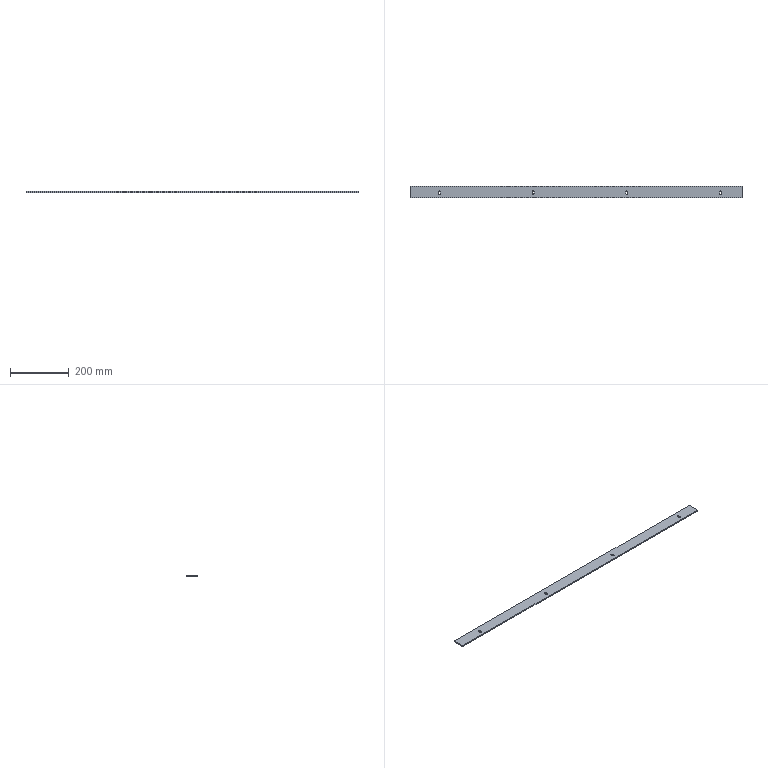Component | SolidWorks | SlideRail-1 | 1 solid | 22 faces | box 1133 x 40 x 4 mm | volume 180104 mm3 | plane 14 | cylinder 8 | commonest cylinder face diameters 7 x8
build123d program:
from build123d import *

# Parameters (mm, degrees)
SKETCH1_W           = 1133
SKETCH1_H           = 40
BOSS_EXTRUDE1_DEPTH = 4
CUT_EXTRUDE1_DEPTH  = 10
LPATTERN1_COUNT     = 4
LPATTERN1_PITCH     = 320


with BuildPart() as part:
    # Sketch1 → Boss-Extrude1 (new body)
    with BuildSketch(Plane.XY):
        with Locations((460.15, 15.317)):
            Rectangle(SKETCH1_W, SKETCH1_H)
    extrude(amount=BOSS_EXTRUDE1_DEPTH)

    # Sketch2 → Cut-Extrude1 (cut)
    with BuildSketch(Plane.XY.offset(4)):
        with BuildLine():
            Line((-2.85, 15.317), (-2.85, 10.317))
            ThreePointArc((-2.85, 10.317), (-6.35, 6.817), (-9.85, 10.317))
            Line((-9.85, 10.317), (-9.85, 15.317))
            ThreePointArc((-9.85, 15.317), (-6.35, 18.817), (-2.85, 15.317))
        make_face()
    cut_extrude1 = extrude(amount=-CUT_EXTRUDE1_DEPTH, mode=Mode.SUBTRACT)

    # LPattern1: Cut-Extrude1 ×4
    with Locations(*[(i * LPATTERN1_PITCH, 0, 0) for i in range(1, LPATTERN1_COUNT)]):
        add(cut_extrude1, mode=Mode.SUBTRACT)


solid = part.part

# Placed as in the assembly
solid = solid.moved(Location((-791.2, -396.75, 487.481), (0, 0, 0)))
STEP:
#1=COLOUR_RGB('',0.7922,0.8196,0.9333);
#2=FILL_AREA_STYLE_COLOUR('',#1);
#3=FILL_AREA_STYLE('',(#2));
#4=SURFACE_STYLE_FILL_AREA(#3);
#5=SURFACE_SIDE_STYLE('',(#4));
#6=SURFACE_STYLE_USAGE(.BOTH.,#5);
#7=PRESENTATION_STYLE_ASSIGNMENT((#6));
#8=CARTESIAN_POINT('',(-35.337,-14.23,19.192));
#9=VERTEX_POINT('',#8);
#10=CARTESIAN_POINT('',(-35.337,-15.804,19.192));
#11=VERTEX_POINT('',#10);
#12=CARTESIAN_POINT('',(-35.337,-14.23,19.192));
#13=DIRECTION('',(0.,-1.,0.));
#14=VECTOR('',#13,39.37);
#15=LINE('',#12,#14);
#16=EDGE_CURVE('',#9,#11,#15,.T.);
#17=ORIENTED_EDGE('',*,*,#16,.T.);
#18=CARTESIAN_POINT('',(-35.337,-15.804,19.35));
#19=VERTEX_POINT('',#18);
#20=CARTESIAN_POINT('',(-35.337,-15.804,19.35));
#21=DIRECTION('',(0.,0.,-1.));
#22=VECTOR('',#21,39.37);
#23=LINE('',#20,#22);
#24=EDGE_CURVE('',#19,#11,#23,.T.);
#25=ORIENTED_EDGE('',*,*,#24,.F.);
#26=CARTESIAN_POINT('',(-35.337,-14.23,19.35));
#27=VERTEX_POINT('',#26);
#28=CARTESIAN_POINT('',(-35.337,-14.23,19.35));
#29=DIRECTION('',(0.,-1.,0.));
#30=VECTOR('',#29,39.37);
#31=LINE('',#28,#30);
#32=EDGE_CURVE('',#27,#19,#31,.T.);
#33=ORIENTED_EDGE('',*,*,#32,.F.);
#34=CARTESIAN_POINT('',(-35.337,-14.23,19.35));
#35=DIRECTION('',(0.,0.,-1.));
#36=VECTOR('',#35,39.37);
#37=LINE('',#34,#36);
#38=EDGE_CURVE('',#27,#9,#37,.T.);
#39=ORIENTED_EDGE('',*,*,#38,.T.);
#40=EDGE_LOOP('',(#17,#25,#33,#39));
#41=FACE_OUTER_BOUND('',#40,.T.);
#42=CARTESIAN_POINT('',(-35.337,-14.23,19.35));
#43=DIRECTION('',(1.,0.,0.));
#44=DIRECTION('',(0.,0.,-1.));
#45=AXIS2_PLACEMENT_3D('',#42,#43,#44);
#46=PLANE('',#45);
#47=ADVANCED_FACE('',(#41),#46,.F.);
#48=CARTESIAN_POINT('',(9.27,-15.804,19.192));
#49=VERTEX_POINT('',#48);
#50=CARTESIAN_POINT('',(-35.337,-15.804,19.192));
#51=DIRECTION('',(1.,-0.,0.));
#52=VECTOR('',#51,39.37);
#53=LINE('',#50,#52);
#54=EDGE_CURVE('',#11,#49,#53,.T.);
#55=ORIENTED_EDGE('',*,*,#54,.T.);
#56=CARTESIAN_POINT('',(9.27,-15.804,19.35));
#57=VERTEX_POINT('',#56);
#58=CARTESIAN_POINT('',(9.27,-15.804,19.35));
#59=DIRECTION('',(0.,0.,-1.));
#60=VECTOR('',#59,39.37);
#61=LINE('',#58,#60);
#62=EDGE_CURVE('',#57,#49,#61,.T.);
#63=ORIENTED_EDGE('',*,*,#62,.F.);
#64=CARTESIAN_POINT('',(-35.337,-15.804,19.35));
#65=DIRECTION('',(1.,-0.,0.));
#66=VECTOR('',#65,39.37);
#67=LINE('',#64,#66);
#68=EDGE_CURVE('',#19,#57,#67,.T.);
#69=ORIENTED_EDGE('',*,*,#68,.F.);
#70=ORIENTED_EDGE('',*,*,#24,.T.);
#71=EDGE_LOOP('',(#55,#63,#69,#70));
#72=FACE_OUTER_BOUND('',#71,.T.);
#73=CARTESIAN_POINT('',(-35.337,-15.804,19.35));
#74=DIRECTION('',(0.,1.,0.));
#75=DIRECTION('',(-1.,0.,0.));
#76=AXIS2_PLACEMENT_3D('',#73,#74,#75);
#77=PLANE('',#76);
#78=ADVANCED_FACE('',(#72),#77,.F.);
#79=CARTESIAN_POINT('',(9.27,-14.23,19.192));
#80=VERTEX_POINT('',#79);
#81=CARTESIAN_POINT('',(9.27,-14.23,19.192));
#82=DIRECTION('',(0.,1.,0.));
#83=VECTOR('',#82,39.37);
#84=LINE('',#81,#83);
#85=EDGE_CURVE('',#49,#80,#84,.T.);
#86=ORIENTED_EDGE('',*,*,#85,.T.);
#87=CARTESIAN_POINT('',(9.27,-14.23,19.35));
#88=VERTEX_POINT('',#87);
#89=CARTESIAN_POINT('',(9.27,-14.23,19.35));
#90=DIRECTION('',(0.,0.,-1.));
#91=VECTOR('',#90,39.37);
#92=LINE('',#89,#91);
#93=EDGE_CURVE('',#88,#80,#92,.T.);
#94=ORIENTED_EDGE('',*,*,#93,.F.);
#95=CARTESIAN_POINT('',(9.27,-14.23,19.35));
#96=DIRECTION('',(0.,1.,0.));
#97=VECTOR('',#96,39.37);
#98=LINE('',#95,#97);
#99=EDGE_CURVE('',#57,#88,#98,.T.);
#100=ORIENTED_EDGE('',*,*,#99,.F.);
#101=ORIENTED_EDGE('',*,*,#62,.T.);
#102=EDGE_LOOP('',(#86,#94,#100,#101));
#103=FACE_OUTER_BOUND('',#102,.T.);
#104=CARTESIAN_POINT('',(9.27,-14.23,19.35));
#105=DIRECTION('',(-1.,0.,0.));
#106=DIRECTION('',(0.,0.,1.));
#107=AXIS2_PLACEMENT_3D('',#104,#105,#106);
#108=PLANE('',#107);
#109=ADVANCED_FACE('',(#103),#108,.F.);
#110=CARTESIAN_POINT('',(-35.337,-14.23,19.192));
#111=DIRECTION('',(-1.,0.,0.));
#112=VECTOR('',#111,39.37);
#113=LINE('',#110,#112);
#114=EDGE_CURVE('',#80,#9,#113,.T.);
#115=ORIENTED_EDGE('',*,*,#114,.T.);
#116=ORIENTED_EDGE('',*,*,#38,.F.);
#117=CARTESIAN_POINT('',(-35.337,-14.23,19.35));
#118=DIRECTION('',(-1.,0.,0.));
#119=VECTOR('',#118,39.37);
#120=LINE('',#117,#119);
#121=EDGE_CURVE('',#88,#27,#120,.T.);
#122=ORIENTED_EDGE('',*,*,#121,.F.);
#123=ORIENTED_EDGE('',*,*,#93,.T.);
#124=EDGE_LOOP('',(#115,#116,#122,#123));
#125=FACE_OUTER_BOUND('',#124,.T.);
#126=CARTESIAN_POINT('',(-35.337,-14.23,19.35));
#127=DIRECTION('',(0.,-1.,0.));
#128=DIRECTION('',(0.,0.,-1.));
#129=AXIS2_PLACEMENT_3D('',#126,#127,#128);
#130=PLANE('',#129);
#131=ADVANCED_FACE('',(#125),#130,.F.);
#132=CARTESIAN_POINT('',(-18.663,-15.017,19.35));
#133=VERTEX_POINT('',#132);
#134=CARTESIAN_POINT('',(-18.939,-15.017,19.35));
#135=VERTEX_POINT('',#134);
#136=CARTESIAN_POINT('',(-18.801,-15.017,19.35));
#137=DIRECTION('',(0.,0.,1.));
#138=DIRECTION('',(1.,0.,0.));
#139=AXIS2_PLACEMENT_3D('',#136,#137,#138);
#140=CIRCLE('',#139,0.1378);
#141=EDGE_CURVE('',#133,#135,#140,.T.);
#142=ORIENTED_EDGE('',*,*,#141,.F.);
#143=CARTESIAN_POINT('',(-18.663,-15.214,19.35));
#144=VERTEX_POINT('',#143);
#145=CARTESIAN_POINT('',(-18.663,-15.017,19.35));
#146=DIRECTION('',(0.,1.,0.));
#147=VECTOR('',#146,39.37);
#148=LINE('',#145,#147);
#149=EDGE_CURVE('',#144,#133,#148,.T.);
#150=ORIENTED_EDGE('',*,*,#149,.F.);
#151=CARTESIAN_POINT('',(-18.939,-15.214,19.35));
#152=VERTEX_POINT('',#151);
#153=CARTESIAN_POINT('',(-18.801,-15.214,19.35));
#154=DIRECTION('',(0.,0.,1.));
#155=DIRECTION('',(1.,0.,0.));
#156=AXIS2_PLACEMENT_3D('',#153,#154,#155);
#157=CIRCLE('',#156,0.1378);
#158=EDGE_CURVE('',#152,#144,#157,.T.);
#159=ORIENTED_EDGE('',*,*,#158,.F.);
#160=CARTESIAN_POINT('',(-18.939,-15.017,19.35));
#161=DIRECTION('',(0.,-1.,0.));
#162=VECTOR('',#161,39.37);
#163=LINE('',#160,#162);
#164=EDGE_CURVE('',#135,#152,#163,.T.);
#165=ORIENTED_EDGE('',*,*,#164,.F.);
#166=EDGE_LOOP('',(#142,#150,#159,#165));
#167=FACE_BOUND('',#166,.T.);
#168=CARTESIAN_POINT('',(-31.262,-15.017,19.35));
#169=VERTEX_POINT('',#168);
#170=CARTESIAN_POINT('',(-31.537,-15.017,19.35));
#171=VERTEX_POINT('',#170);
#172=CARTESIAN_POINT('',(-31.4,-15.017,19.35));
#173=DIRECTION('',(0.,0.,1.));
#174=DIRECTION('',(1.,0.,0.));
#175=AXIS2_PLACEMENT_3D('',#172,#173,#174);
#176=CIRCLE('',#175,0.1378);
#177=EDGE_CURVE('',#169,#171,#176,.T.);
#178=ORIENTED_EDGE('',*,*,#177,.F.);
#179=CARTESIAN_POINT('',(-31.262,-15.214,19.35));
#180=VERTEX_POINT('',#179);
#181=CARTESIAN_POINT('',(-31.262,-15.017,19.35));
#182=DIRECTION('',(0.,1.,0.));
#183=VECTOR('',#182,39.37);
#184=LINE('',#181,#183);
#185=EDGE_CURVE('',#180,#169,#184,.T.);
#186=ORIENTED_EDGE('',*,*,#185,.F.);
#187=CARTESIAN_POINT('',(-31.537,-15.214,19.35));
#188=VERTEX_POINT('',#187);
#189=CARTESIAN_POINT('',(-31.4,-15.214,19.35));
#190=DIRECTION('',(0.,0.,1.));
#191=DIRECTION('',(1.,0.,0.));
#192=AXIS2_PLACEMENT_3D('',#189,#190,#191);
#193=CIRCLE('',#192,0.1378);
#194=EDGE_CURVE('',#188,#180,#193,.T.);
#195=ORIENTED_EDGE('',*,*,#194,.F.);
#196=CARTESIAN_POINT('',(-31.537,-15.017,19.35));
#197=DIRECTION('',(0.,-1.,0.));
#198=VECTOR('',#197,39.37);
#199=LINE('',#196,#198);
#200=EDGE_CURVE('',#171,#188,#199,.T.);
#201=ORIENTED_EDGE('',*,*,#200,.F.);
#202=EDGE_LOOP('',(#178,#186,#195,#201));
#203=FACE_BOUND('',#202,.T.);
#204=ORIENTED_EDGE('',*,*,#32,.T.);
#205=ORIENTED_EDGE('',*,*,#68,.T.);
#206=ORIENTED_EDGE('',*,*,#99,.T.);
#207=ORIENTED_EDGE('',*,*,#121,.T.);
#208=EDGE_LOOP('',(#204,#205,#206,#207));
#209=FACE_OUTER_BOUND('',#208,.T.);
#210=CARTESIAN_POINT('',(-6.065,-15.017,19.35));
#211=VERTEX_POINT('',#210);
#212=CARTESIAN_POINT('',(-6.341,-15.017,19.35));
#213=VERTEX_POINT('',#212);
#214=CARTESIAN_POINT('',(-6.203,-15.017,19.35));
#215=DIRECTION('',(0.,0.,1.));
#216=DIRECTION('',(1.,0.,0.));
#217=AXIS2_PLACEMENT_3D('',#214,#215,#216);
#218=CIRCLE('',#217,0.1378);
#219=EDGE_CURVE('',#211,#213,#218,.T.);
#220=ORIENTED_EDGE('',*,*,#219,.F.);
#221=CARTESIAN_POINT('',(-6.065,-15.214,19.35));
#222=VERTEX_POINT('',#221);
#223=CARTESIAN_POINT('',(-6.065,-15.017,19.35));
#224=DIRECTION('',(0.,1.,0.));
#225=VECTOR('',#224,39.37);
#226=LINE('',#223,#225);
#227=EDGE_CURVE('',#222,#211,#226,.T.);
#228=ORIENTED_EDGE('',*,*,#227,.F.);
#229=CARTESIAN_POINT('',(-6.341,-15.214,19.35));
#230=VERTEX_POINT('',#229);
#231=CARTESIAN_POINT('',(-6.203,-15.214,19.35));
#232=DIRECTION('',(0.,0.,1.));
#233=DIRECTION('',(1.,0.,0.));
#234=AXIS2_PLACEMENT_3D('',#231,#232,#233);
#235=CIRCLE('',#234,0.1378);
#236=EDGE_CURVE('',#230,#222,#235,.T.);
#237=ORIENTED_EDGE('',*,*,#236,.F.);
#238=CARTESIAN_POINT('',(-6.341,-15.017,19.35));
#239=DIRECTION('',(0.,-1.,0.));
#240=VECTOR('',#239,39.37);
#241=LINE('',#238,#240);
#242=EDGE_CURVE('',#213,#230,#241,.T.);
#243=ORIENTED_EDGE('',*,*,#242,.F.);
#244=EDGE_LOOP('',(#220,#228,#237,#243));
#245=FACE_BOUND('',#244,.T.);
#246=CARTESIAN_POINT('',(6.533,-15.017,19.35));
#247=VERTEX_POINT('',#246);
#248=CARTESIAN_POINT('',(6.258,-15.017,19.35));
#249=VERTEX_POINT('',#248);
#250=CARTESIAN_POINT('',(6.396,-15.017,19.35));
#251=DIRECTION('',(0.,0.,1.));
#252=DIRECTION('',(1.,0.,0.));
#253=AXIS2_PLACEMENT_3D('',#250,#251,#252);
#254=CIRCLE('',#253,0.1378);
#255=EDGE_CURVE('',#247,#249,#254,.T.);
#256=ORIENTED_EDGE('',*,*,#255,.F.);
#257=CARTESIAN_POINT('',(6.533,-15.214,19.35));
#258=VERTEX_POINT('',#257);
#259=CARTESIAN_POINT('',(6.533,-15.017,19.35));
#260=DIRECTION('',(0.,1.,0.));
#261=VECTOR('',#260,39.37);
#262=LINE('',#259,#261);
#263=EDGE_CURVE('',#258,#247,#262,.T.);
#264=ORIENTED_EDGE('',*,*,#263,.F.);
#265=CARTESIAN_POINT('',(6.258,-15.214,19.35));
#266=VERTEX_POINT('',#265);
#267=CARTESIAN_POINT('',(6.396,-15.214,19.35));
#268=DIRECTION('',(0.,0.,1.));
#269=DIRECTION('',(1.,0.,0.));
#270=AXIS2_PLACEMENT_3D('',#267,#268,#269);
#271=CIRCLE('',#270,0.1378);
#272=EDGE_CURVE('',#266,#258,#271,.T.);
#273=ORIENTED_EDGE('',*,*,#272,.F.);
#274=CARTESIAN_POINT('',(6.258,-15.017,19.35));
#275=DIRECTION('',(0.,-1.,0.));
#276=VECTOR('',#275,39.37);
#277=LINE('',#274,#276);
#278=EDGE_CURVE('',#249,#266,#277,.T.);
#279=ORIENTED_EDGE('',*,*,#278,.F.);
#280=EDGE_LOOP('',(#256,#264,#273,#279));
#281=FACE_BOUND('',#280,.T.);
#282=CARTESIAN_POINT('',(-31.15,-15.62,19.35));
#283=DIRECTION('',(0.,0.,1.));
#284=DIRECTION('',(1.,0.,0.));
#285=AXIS2_PLACEMENT_3D('',#282,#283,#284);
#286=PLANE('',#285);
#287=ADVANCED_FACE('',(#167,#203,#209,#245,#281),#286,.T.);
#288=CARTESIAN_POINT('',(-18.663,-15.214,19.192));
#289=VERTEX_POINT('',#288);
#290=CARTESIAN_POINT('',(-18.663,-15.017,19.192));
#291=VERTEX_POINT('',#290);
#292=CARTESIAN_POINT('',(-18.663,-15.62,19.192));
#293=DIRECTION('',(0.,1.,0.));
#294=VECTOR('',#293,39.37);
#295=LINE('',#292,#294);
#296=EDGE_CURVE('',#289,#291,#295,.T.);
#297=ORIENTED_EDGE('',*,*,#296,.T.);
#298=CARTESIAN_POINT('',(-18.939,-15.017,19.192));
#299=VERTEX_POINT('',#298);
#300=CARTESIAN_POINT('',(-18.801,-15.017,19.192));
#301=DIRECTION('',(0.,0.,1.));
#302=DIRECTION('',(1.,0.,0.));
#303=AXIS2_PLACEMENT_3D('',#300,#301,#302);
#304=CIRCLE('',#303,0.1378);
#305=EDGE_CURVE('',#291,#299,#304,.T.);
#306=ORIENTED_EDGE('',*,*,#305,.T.);
#307=CARTESIAN_POINT('',(-18.939,-15.214,19.192));
#308=VERTEX_POINT('',#307);
#309=CARTESIAN_POINT('',(-18.939,-15.62,19.192));
#310=DIRECTION('',(0.,-1.,0.));
#311=VECTOR('',#310,39.37);
#312=LINE('',#309,#311);
#313=EDGE_CURVE('',#299,#308,#312,.T.);
#314=ORIENTED_EDGE('',*,*,#313,.T.);
#315=CARTESIAN_POINT('',(-18.801,-15.214,19.192));
#316=DIRECTION('',(0.,0.,1.));
#317=DIRECTION('',(1.,0.,0.));
#318=AXIS2_PLACEMENT_3D('',#315,#316,#317);
#319=CIRCLE('',#318,0.1378);
#320=EDGE_CURVE('',#308,#289,#319,.T.);
#321=ORIENTED_EDGE('',*,*,#320,.T.);
#322=EDGE_LOOP('',(#297,#306,#314,#321));
#323=FACE_BOUND('',#322,.T.);
#324=CARTESIAN_POINT('',(-31.262,-15.214,19.192));
#325=VERTEX_POINT('',#324);
#326=CARTESIAN_POINT('',(-31.262,-15.017,19.192));
#327=VERTEX_POINT('',#326);
#328=CARTESIAN_POINT('',(-31.262,-15.62,19.192));
#329=DIRECTION('',(0.,1.,0.));
#330=VECTOR('',#329,39.37);
#331=LINE('',#328,#330);
#332=EDGE_CURVE('',#325,#327,#331,.T.);
#333=ORIENTED_EDGE('',*,*,#332,.T.);
#334=CARTESIAN_POINT('',(-31.537,-15.017,19.192));
#335=VERTEX_POINT('',#334);
#336=CARTESIAN_POINT('',(-31.4,-15.017,19.192));
#337=DIRECTION('',(0.,0.,1.));
#338=DIRECTION('',(1.,0.,0.));
#339=AXIS2_PLACEMENT_3D('',#336,#337,#338);
#340=CIRCLE('',#339,0.1378);
#341=EDGE_CURVE('',#327,#335,#340,.T.);
#342=ORIENTED_EDGE('',*,*,#341,.T.);
#343=CARTESIAN_POINT('',(-31.537,-15.214,19.192));
#344=VERTEX_POINT('',#343);
#345=CARTESIAN_POINT('',(-31.537,-15.62,19.192));
#346=DIRECTION('',(0.,-1.,0.));
#347=VECTOR('',#346,39.37);
#348=LINE('',#345,#347);
#349=EDGE_CURVE('',#335,#344,#348,.T.);
#350=ORIENTED_EDGE('',*,*,#349,.T.);
#351=CARTESIAN_POINT('',(-31.4,-15.214,19.192));
#352=DIRECTION('',(0.,0.,1.));
#353=DIRECTION('',(1.,0.,0.));
#354=AXIS2_PLACEMENT_3D('',#351,#352,#353);
#355=CIRCLE('',#354,0.1378);
#356=EDGE_CURVE('',#344,#325,#355,.T.);
#357=ORIENTED_EDGE('',*,*,#356,.T.);
#358=EDGE_LOOP('',(#333,#342,#350,#357));
#359=FACE_BOUND('',#358,.T.);
#360=ORIENTED_EDGE('',*,*,#16,.F.);
#361=ORIENTED_EDGE('',*,*,#114,.F.);
#362=ORIENTED_EDGE('',*,*,#85,.F.);
#363=ORIENTED_EDGE('',*,*,#54,.F.);
#364=EDGE_LOOP('',(#360,#361,#362,#363));
#365=FACE_OUTER_BOUND('',#364,.T.);
#366=CARTESIAN_POINT('',(-6.065,-15.017,19.192));
#367=VERTEX_POINT('',#366);
#368=CARTESIAN_POINT('',(-6.341,-15.017,19.192));
#369=VERTEX_POINT('',#368);
#370=CARTESIAN_POINT('',(-6.203,-15.017,19.192));
#371=DIRECTION('',(0.,0.,1.));
#372=DIRECTION('',(1.,0.,0.));
#373=AXIS2_PLACEMENT_3D('',#370,#371,#372);
#374=CIRCLE('',#373,0.1378);
#375=EDGE_CURVE('',#367,#369,#374,.T.);
#376=ORIENTED_EDGE('',*,*,#375,.T.);
#377=CARTESIAN_POINT('',(-6.341,-15.214,19.192));
#378=VERTEX_POINT('',#377);
#379=CARTESIAN_POINT('',(-6.341,-15.62,19.192));
#380=DIRECTION('',(0.,-1.,0.));
#381=VECTOR('',#380,39.37);
#382=LINE('',#379,#381);
#383=EDGE_CURVE('',#369,#378,#382,.T.);
#384=ORIENTED_EDGE('',*,*,#383,.T.);
#385=CARTESIAN_POINT('',(-6.065,-15.214,19.192));
#386=VERTEX_POINT('',#385);
#387=CARTESIAN_POINT('',(-6.203,-15.214,19.192));
#388=DIRECTION('',(0.,0.,1.));
#389=DIRECTION('',(1.,0.,0.));
#390=AXIS2_PLACEMENT_3D('',#387,#388,#389);
#391=CIRCLE('',#390,0.1378);
#392=EDGE_CURVE('',#378,#386,#391,.T.);
#393=ORIENTED_EDGE('',*,*,#392,.T.);
#394=CARTESIAN_POINT('',(-6.065,-15.62,19.192));
#395=DIRECTION('',(0.,1.,0.));
#396=VECTOR('',#395,39.37);
#397=LINE('',#394,#396);
#398=EDGE_CURVE('',#386,#367,#397,.T.);
#399=ORIENTED_EDGE('',*,*,#398,.T.);
#400=EDGE_LOOP('',(#376,#384,#393,#399));
#401=FACE_BOUND('',#400,.T.);
#402=CARTESIAN_POINT('',(6.533,-15.017,19.192));
#403=VERTEX_POINT('',#402);
#404=CARTESIAN_POINT('',(6.258,-15.017,19.192));
#405=VERTEX_POINT('',#404);
#406=CARTESIAN_POINT('',(6.396,-15.017,19.192));
#407=DIRECTION('',(0.,0.,1.));
#408=DIRECTION('',(1.,0.,0.));
#409=AXIS2_PLACEMENT_3D('',#406,#407,#408);
#410=CIRCLE('',#409,0.1378);
#411=EDGE_CURVE('',#403,#405,#410,.T.);
#412=ORIENTED_EDGE('',*,*,#411,.T.);
#413=CARTESIAN_POINT('',(6.258,-15.214,19.192));
#414=VERTEX_POINT('',#413);
#415=CARTESIAN_POINT('',(6.258,-15.62,19.192));
#416=DIRECTION('',(0.,-1.,0.));
#417=VECTOR('',#416,39.37);
#418=LINE('',#415,#417);
#419=EDGE_CURVE('',#405,#414,#418,.T.);
#420=ORIENTED_EDGE('',*,*,#419,.T.);
#421=CARTESIAN_POINT('',(6.533,-15.214,19.192));
#422=VERTEX_POINT('',#421);
#423=CARTESIAN_POINT('',(6.396,-15.214,19.192));
#424=DIRECTION('',(0.,0.,1.));
#425=DIRECTION('',(1.,0.,0.));
#426=AXIS2_PLACEMENT_3D('',#423,#424,#425);
#427=CIRCLE('',#426,0.1378);
#428=EDGE_CURVE('',#414,#422,#427,.T.);
#429=ORIENTED_EDGE('',*,*,#428,.T.);
#430=CARTESIAN_POINT('',(6.533,-15.62,19.192));
#431=DIRECTION('',(0.,1.,0.));
#432=VECTOR('',#431,39.37);
#433=LINE('',#430,#432);
#434=EDGE_CURVE('',#422,#403,#433,.T.);
#435=ORIENTED_EDGE('',*,*,#434,.T.);
#436=EDGE_LOOP('',(#412,#420,#429,#435));
#437=FACE_BOUND('',#436,.T.);
#438=CARTESIAN_POINT('',(-31.15,-15.62,19.192));
#439=DIRECTION('',(0.,0.,1.));
#440=DIRECTION('',(1.,0.,0.));
#441=AXIS2_PLACEMENT_3D('',#438,#439,#440);
#442=PLANE('',#441);
#443=ADVANCED_FACE('',(#323,#359,#365,#401,#437),#442,.F.);
#444=CARTESIAN_POINT('',(-31.262,-15.017,18.956));
#445=DIRECTION('',(0.,0.,1.));
#446=VECTOR('',#445,39.37);
#447=LINE('',#444,#446);
#448=EDGE_CURVE('',#327,#169,#447,.T.);
#449=ORIENTED_EDGE('',*,*,#448,.T.);
#450=ORIENTED_EDGE('',*,*,#177,.T.);
#451=CARTESIAN_POINT('',(-31.537,-15.017,18.956));
#452=DIRECTION('',(0.,0.,1.));
#453=VECTOR('',#452,39.37);
#454=LINE('',#451,#453);
#455=EDGE_CURVE('',#335,#171,#454,.T.);
#456=ORIENTED_EDGE('',*,*,#455,.F.);
#457=ORIENTED_EDGE('',*,*,#341,.F.);
#458=EDGE_LOOP('',(#449,#450,#456,#457));
#459=FACE_OUTER_BOUND('',#458,.T.);
#460=CARTESIAN_POINT('',(-31.4,-15.017,18.956));
#461=DIRECTION('',(0.,0.,1.));
#462=DIRECTION('',(1.,0.,0.));
#463=AXIS2_PLACEMENT_3D('',#460,#461,#462);
#464=CYLINDRICAL_SURFACE('',#463,0.1378);
#465=ADVANCED_FACE('',(#459),#464,.F.);
#466=CARTESIAN_POINT('',(-31.262,-15.214,18.956));
#467=DIRECTION('',(0.,0.,1.));
#468=VECTOR('',#467,39.37);
#469=LINE('',#466,#468);
#470=EDGE_CURVE('',#325,#180,#469,.T.);
#471=ORIENTED_EDGE('',*,*,#470,.T.);
#472=ORIENTED_EDGE('',*,*,#185,.T.);
#473=ORIENTED_EDGE('',*,*,#448,.F.);
#474=ORIENTED_EDGE('',*,*,#332,.F.);
#475=EDGE_LOOP('',(#471,#472,#473,#474));
#476=FACE_OUTER_BOUND('',#475,.T.);
#477=CARTESIAN_POINT('',(-31.262,-15.017,18.956));
#478=DIRECTION('',(1.,0.,0.));
#479=DIRECTION('',(0.,0.,-1.));
#480=AXIS2_PLACEMENT_3D('',#477,#478,#479);
#481=PLANE('',#480);
#482=ADVANCED_FACE('',(#476),#481,.F.);
#483=CARTESIAN_POINT('',(-31.537,-15.214,18.956));
#484=DIRECTION('',(0.,0.,1.));
#485=VECTOR('',#484,39.37);
#486=LINE('',#483,#485);
#487=EDGE_CURVE('',#344,#188,#486,.T.);
#488=ORIENTED_EDGE('',*,*,#487,.T.);
#489=ORIENTED_EDGE('',*,*,#194,.T.);
#490=ORIENTED_EDGE('',*,*,#470,.F.);
#491=ORIENTED_EDGE('',*,*,#356,.F.);
#492=EDGE_LOOP('',(#488,#489,#490,#491));
#493=FACE_OUTER_BOUND('',#492,.T.);
#494=CARTESIAN_POINT('',(-31.4,-15.214,18.956));
#495=DIRECTION('',(0.,0.,1.));
#496=DIRECTION('',(1.,0.,0.));
#497=AXIS2_PLACEMENT_3D('',#494,#495,#496);
#498=CYLINDRICAL_SURFACE('',#497,0.1378);
#499=ADVANCED_FACE('',(#493),#498,.F.);
#500=ORIENTED_EDGE('',*,*,#455,.T.);
#501=ORIENTED_EDGE('',*,*,#200,.T.);
#502=ORIENTED_EDGE('',*,*,#487,.F.);
#503=ORIENTED_EDGE('',*,*,#349,.F.);
#504=EDGE_LOOP('',(#500,#501,#502,#503));
#505=FACE_OUTER_BOUND('',#504,.T.);
#506=CARTESIAN_POINT('',(-31.537,-15.017,18.956));
#507=DIRECTION('',(-1.,-0.,0.));
#508=DIRECTION('',(0.,-1.,0.));
#509=AXIS2_PLACEMENT_3D('',#506,#507,#508);
#510=PLANE('',#509);
#511=ADVANCED_FACE('',(#505),#510,.F.);
#512=CARTESIAN_POINT('',(-18.663,-15.017,18.956));
#513=DIRECTION('',(0.,0.,1.));
#514=VECTOR('',#513,39.37);
#515=LINE('',#512,#514);
#516=EDGE_CURVE('',#291,#133,#515,.T.);
#517=ORIENTED_EDGE('',*,*,#516,.T.);
#518=ORIENTED_EDGE('',*,*,#141,.T.);
#519=CARTESIAN_POINT('',(-18.939,-15.017,18.956));
#520=DIRECTION('',(0.,0.,1.));
#521=VECTOR('',#520,39.37);
#522=LINE('',#519,#521);
#523=EDGE_CURVE('',#299,#135,#522,.T.);
#524=ORIENTED_EDGE('',*,*,#523,.F.);
#525=ORIENTED_EDGE('',*,*,#305,.F.);
#526=EDGE_LOOP('',(#517,#518,#524,#525));
#527=FACE_OUTER_BOUND('',#526,.T.);
#528=CARTESIAN_POINT('',(-18.801,-15.017,18.956));
#529=DIRECTION('',(0.,0.,1.));
#530=DIRECTION('',(1.,0.,0.));
#531=AXIS2_PLACEMENT_3D('',#528,#529,#530);
#532=CYLINDRICAL_SURFACE('',#531,0.1378);
#533=ADVANCED_FACE('',(#527),#532,.F.);
#534=CARTESIAN_POINT('',(-18.663,-15.214,18.956));
#535=DIRECTION('',(0.,0.,1.));
#536=VECTOR('',#535,39.37);
#537=LINE('',#534,#536);
#538=EDGE_CURVE('',#289,#144,#537,.T.);
#539=ORIENTED_EDGE('',*,*,#538,.T.);
#540=ORIENTED_EDGE('',*,*,#149,.T.);
#541=ORIENTED_EDGE('',*,*,#516,.F.);
#542=ORIENTED_EDGE('',*,*,#296,.F.);
#543=EDGE_LOOP('',(#539,#540,#541,#542));
#544=FACE_OUTER_BOUND('',#543,.T.);
#545=CARTESIAN_POINT('',(-18.663,-15.017,18.956));
#546=DIRECTION('',(1.,0.,0.));
#547=DIRECTION('',(0.,0.,-1.));
#548=AXIS2_PLACEMENT_3D('',#545,#546,#547);
#549=PLANE('',#548);
#550=ADVANCED_FACE('',(#544),#549,.F.);
#551=CARTESIAN_POINT('',(-18.939,-15.214,18.956));
#552=DIRECTION('',(0.,0.,1.));
#553=VECTOR('',#552,39.37);
#554=LINE('',#551,#553);
#555=EDGE_CURVE('',#308,#152,#554,.T.);
#556=ORIENTED_EDGE('',*,*,#555,.T.);
#557=ORIENTED_EDGE('',*,*,#158,.T.);
#558=ORIENTED_EDGE('',*,*,#538,.F.);
#559=ORIENTED_EDGE('',*,*,#320,.F.);
#560=EDGE_LOOP('',(#556,#557,#558,#559));
#561=FACE_OUTER_BOUND('',#560,.T.);
#562=CARTESIAN_POINT('',(-18.801,-15.214,18.956));
#563=DIRECTION('',(0.,0.,1.));
#564=DIRECTION('',(1.,0.,0.));
#565=AXIS2_PLACEMENT_3D('',#562,#563,#564);
#566=CYLINDRICAL_SURFACE('',#565,0.1378);
#567=ADVANCED_FACE('',(#561),#566,.F.);
#568=ORIENTED_EDGE('',*,*,#523,.T.);
#569=ORIENTED_EDGE('',*,*,#164,.T.);
#570=ORIENTED_EDGE('',*,*,#555,.F.);
#571=ORIENTED_EDGE('',*,*,#313,.F.);
#572=EDGE_LOOP('',(#568,#569,#570,#571));
#573=FACE_OUTER_BOUND('',#572,.T.);
#574=CARTESIAN_POINT('',(-18.939,-15.017,18.956));
#575=DIRECTION('',(-1.,-0.,0.));
#576=DIRECTION('',(0.,-1.,0.));
#577=AXIS2_PLACEMENT_3D('',#574,#575,#576);
#578=PLANE('',#577);
#579=ADVANCED_FACE('',(#573),#578,.F.);
#580=CARTESIAN_POINT('',(-6.341,-15.017,18.956));
#581=DIRECTION('',(0.,0.,1.));
#582=VECTOR('',#581,39.37);
#583=LINE('',#580,#582);
#584=EDGE_CURVE('',#369,#213,#583,.T.);
#585=ORIENTED_EDGE('',*,*,#584,.T.);
#586=ORIENTED_EDGE('',*,*,#242,.T.);
#587=CARTESIAN_POINT('',(-6.341,-15.214,18.956));
#588=DIRECTION('',(0.,0.,1.));
#589=VECTOR('',#588,39.37);
#590=LINE('',#587,#589);
#591=EDGE_CURVE('',#378,#230,#590,.T.);
#592=ORIENTED_EDGE('',*,*,#591,.F.);
#593=ORIENTED_EDGE('',*,*,#383,.F.);
#594=EDGE_LOOP('',(#585,#586,#592,#593));
#595=FACE_OUTER_BOUND('',#594,.T.);
#596=CARTESIAN_POINT('',(-6.341,-15.017,18.956));
#597=DIRECTION('',(-1.,-0.,0.));
#598=DIRECTION('',(0.,-1.,0.));
#599=AXIS2_PLACEMENT_3D('',#596,#597,#598);
#600=PLANE('',#599);
#601=ADVANCED_FACE('',(#595),#600,.F.);
#602=ORIENTED_EDGE('',*,*,#591,.T.);
#603=ORIENTED_EDGE('',*,*,#236,.T.);
#604=CARTESIAN_POINT('',(-6.065,-15.214,18.956));
#605=DIRECTION('',(0.,0.,1.));
#606=VECTOR('',#605,39.37);
#607=LINE('',#604,#606);
#608=EDGE_CURVE('',#386,#222,#607,.T.);
#609=ORIENTED_EDGE('',*,*,#608,.F.);
#610=ORIENTED_EDGE('',*,*,#392,.F.);
#611=EDGE_LOOP('',(#602,#603,#609,#610));
#612=FACE_OUTER_BOUND('',#611,.T.);
#613=CARTESIAN_POINT('',(-6.203,-15.214,18.956));
#614=DIRECTION('',(0.,0.,1.));
#615=DIRECTION('',(1.,0.,0.));
#616=AXIS2_PLACEMENT_3D('',#613,#614,#615);
#617=CYLINDRICAL_SURFACE('',#616,0.1378);
#618=ADVANCED_FACE('',(#612),#617,.F.);
#619=ORIENTED_EDGE('',*,*,#608,.T.);
#620=ORIENTED_EDGE('',*,*,#227,.T.);
#621=CARTESIAN_POINT('',(-6.065,-15.017,18.956));
#622=DIRECTION('',(0.,0.,1.));
#623=VECTOR('',#622,39.37);
#624=LINE('',#621,#623);
#625=EDGE_CURVE('',#367,#211,#624,.T.);
#626=ORIENTED_EDGE('',*,*,#625,.F.);
#627=ORIENTED_EDGE('',*,*,#398,.F.);
#628=EDGE_LOOP('',(#619,#620,#626,#627));
#629=FACE_OUTER_BOUND('',#628,.T.);
#630=CARTESIAN_POINT('',(-6.065,-15.017,18.956));
#631=DIRECTION('',(1.,0.,0.));
#632=DIRECTION('',(0.,0.,-1.));
#633=AXIS2_PLACEMENT_3D('',#630,#631,#632);
#634=PLANE('',#633);
#635=ADVANCED_FACE('',(#629),#634,.F.);
#636=ORIENTED_EDGE('',*,*,#625,.T.);
#637=ORIENTED_EDGE('',*,*,#219,.T.);
#638=ORIENTED_EDGE('',*,*,#584,.F.);
#639=ORIENTED_EDGE('',*,*,#375,.F.);
#640=EDGE_LOOP('',(#636,#637,#638,#639));
#641=FACE_OUTER_BOUND('',#640,.T.);
#642=CARTESIAN_POINT('',(-6.203,-15.017,18.956));
#643=DIRECTION('',(0.,0.,1.));
#644=DIRECTION('',(1.,0.,0.));
#645=AXIS2_PLACEMENT_3D('',#642,#643,#644);
#646=CYLINDRICAL_SURFACE('',#645,0.1378);
#647=ADVANCED_FACE('',(#641),#646,.F.);
#648=CARTESIAN_POINT('',(6.258,-15.017,18.956));
#649=DIRECTION('',(0.,0.,1.));
#650=VECTOR('',#649,39.37);
#651=LINE('',#648,#650);
#652=EDGE_CURVE('',#405,#249,#651,.T.);
#653=ORIENTED_EDGE('',*,*,#652,.T.);
#654=ORIENTED_EDGE('',*,*,#278,.T.);
#655=CARTESIAN_POINT('',(6.258,-15.214,18.956));
#656=DIRECTION('',(0.,0.,1.));
#657=VECTOR('',#656,39.37);
#658=LINE('',#655,#657);
#659=EDGE_CURVE('',#414,#266,#658,.T.);
#660=ORIENTED_EDGE('',*,*,#659,.F.);
#661=ORIENTED_EDGE('',*,*,#419,.F.);
#662=EDGE_LOOP('',(#653,#654,#660,#661));
#663=FACE_OUTER_BOUND('',#662,.T.);
#664=CARTESIAN_POINT('',(6.258,-15.017,18.956));
#665=DIRECTION('',(-1.,-0.,0.));
#666=DIRECTION('',(0.,-1.,0.));
#667=AXIS2_PLACEMENT_3D('',#664,#665,#666);
#668=PLANE('',#667);
#669=ADVANCED_FACE('',(#663),#668,.F.);
#670=ORIENTED_EDGE('',*,*,#659,.T.);
#671=ORIENTED_EDGE('',*,*,#272,.T.);
#672=CARTESIAN_POINT('',(6.533,-15.214,18.956));
#673=DIRECTION('',(0.,0.,1.));
#674=VECTOR('',#673,39.37);
#675=LINE('',#672,#674);
#676=EDGE_CURVE('',#422,#258,#675,.T.);
#677=ORIENTED_EDGE('',*,*,#676,.F.);
#678=ORIENTED_EDGE('',*,*,#428,.F.);
#679=EDGE_LOOP('',(#670,#671,#677,#678));
#680=FACE_OUTER_BOUND('',#679,.T.);
#681=CARTESIAN_POINT('',(6.396,-15.214,18.956));
#682=DIRECTION('',(0.,0.,1.));
#683=DIRECTION('',(1.,0.,0.));
#684=AXIS2_PLACEMENT_3D('',#681,#682,#683);
#685=CYLINDRICAL_SURFACE('',#684,0.1378);
#686=ADVANCED_FACE('',(#680),#685,.F.);
#687=ORIENTED_EDGE('',*,*,#676,.T.);
#688=ORIENTED_EDGE('',*,*,#263,.T.);
#689=CARTESIAN_POINT('',(6.533,-15.017,18.956));
#690=DIRECTION('',(0.,0.,1.));
#691=VECTOR('',#690,39.37);
#692=LINE('',#689,#691);
#693=EDGE_CURVE('',#403,#247,#692,.T.);
#694=ORIENTED_EDGE('',*,*,#693,.F.);
#695=ORIENTED_EDGE('',*,*,#434,.F.);
#696=EDGE_LOOP('',(#687,#688,#694,#695));
#697=FACE_OUTER_BOUND('',#696,.T.);
#698=CARTESIAN_POINT('',(6.533,-15.017,18.956));
#699=DIRECTION('',(1.,0.,0.));
#700=DIRECTION('',(0.,0.,-1.));
#701=AXIS2_PLACEMENT_3D('',#698,#699,#700);
#702=PLANE('',#701);
#703=ADVANCED_FACE('',(#697),#702,.F.);
#704=ORIENTED_EDGE('',*,*,#693,.T.);
#705=ORIENTED_EDGE('',*,*,#255,.T.);
#706=ORIENTED_EDGE('',*,*,#652,.F.);
#707=ORIENTED_EDGE('',*,*,#411,.F.);
#708=EDGE_LOOP('',(#704,#705,#706,#707));
#709=FACE_OUTER_BOUND('',#708,.T.);
#710=CARTESIAN_POINT('',(6.396,-15.017,18.956));
#711=DIRECTION('',(0.,0.,1.));
#712=DIRECTION('',(1.,0.,0.));
#713=AXIS2_PLACEMENT_3D('',#710,#711,#712);
#714=CYLINDRICAL_SURFACE('',#713,0.1378);
#715=ADVANCED_FACE('',(#709),#714,.F.);
#716=CLOSED_SHELL('',(#47,#78,#109,#131,#287,#443,#465,#482,#499,#511,#533,#550,#567,#579,#601,#618,#635,#647,#669,#686,#703,#715));
#717=MANIFOLD_SOLID_BREP('',#716);
#718=STYLED_ITEM('',(#7),#717);
#719=(LENGTH_UNIT()NAMED_UNIT(*)SI_UNIT($,.METRE.));
#720=LENGTH_MEASURE_WITH_UNIT(LENGTH_MEASURE(0.0254),#719);
#721=DIMENSIONAL_EXPONENTS(1.,0.,0.,0.,0.,0.,0.);
#722=(CONVERSION_BASED_UNIT('',#720)LENGTH_UNIT()NAMED_UNIT(#721));
#723=UNCERTAINTY_MEASURE_WITH_UNIT(LENGTH_MEASURE(0.00001),#722,'','');
#724=(NAMED_UNIT(*)PLANE_ANGLE_UNIT()SI_UNIT($,.RADIAN.));
#725=(NAMED_UNIT(*)SI_UNIT($,.STERADIAN.)SOLID_ANGLE_UNIT());
#726=(GEOMETRIC_REPRESENTATION_CONTEXT(3)GLOBAL_UNCERTAINTY_ASSIGNED_CONTEXT((#723))GLOBAL_UNIT_ASSIGNED_CONTEXT((#722,#724,#725))REPRESENTATION_CONTEXT('',''));
#727=MECHANICAL_DESIGN_GEOMETRIC_PRESENTATION_REPRESENTATION('',(#718),#726);
#728=CARTESIAN_POINT('',(0.,0.,0.));
#729=DIRECTION('',(0.,0.,1.));
#730=DIRECTION('',(1.,0.,0.));
#731=AXIS2_PLACEMENT_3D('',#728,#729,#730);
#732=(LENGTH_UNIT()NAMED_UNIT(*)SI_UNIT($,.METRE.));
#733=LENGTH_MEASURE_WITH_UNIT(LENGTH_MEASURE(0.0254),#732);
#734=DIMENSIONAL_EXPONENTS(1.,0.,0.,0.,0.,0.,0.);
#735=(CONVERSION_BASED_UNIT('',#733)LENGTH_UNIT()NAMED_UNIT(#734));
#736=UNCERTAINTY_MEASURE_WITH_UNIT(LENGTH_MEASURE(0.00001),#735,'','');
#737=(NAMED_UNIT(*)PLANE_ANGLE_UNIT()SI_UNIT($,.RADIAN.));
#738=(NAMED_UNIT(*)SI_UNIT($,.STERADIAN.)SOLID_ANGLE_UNIT());
#739=(GEOMETRIC_REPRESENTATION_CONTEXT(3)GLOBAL_UNCERTAINTY_ASSIGNED_CONTEXT((#736))GLOBAL_UNIT_ASSIGNED_CONTEXT((#735,#737,#738))REPRESENTATION_CONTEXT('',''));
#740=ADVANCED_BREP_SHAPE_REPRESENTATION('',(#717,#731),#739);
#741=PRESENTATION_LAYER_ASSIGNMENT('','',(#718));